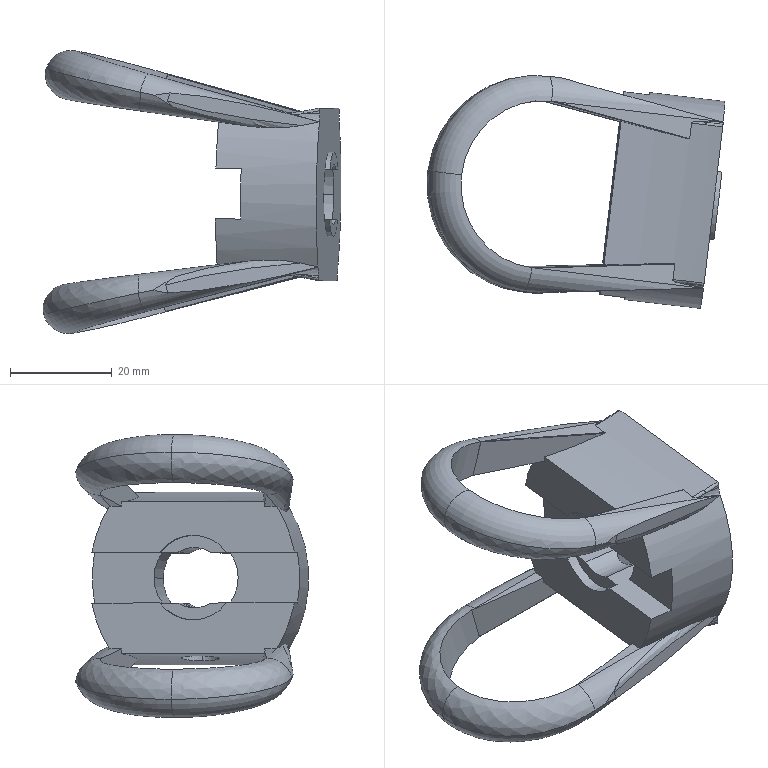Component | SolidWorks | jiazi1-1 | 1 solid | 102 faces | volume 25201 mm3 | cylinder 43 | plane 39 | spline 12 | torus 8 | commonest cylinder face diameters 10 x10 16.68 x7 33 x4 6 x4 43 x4 0.2 x4 54 x3 11.914 x3